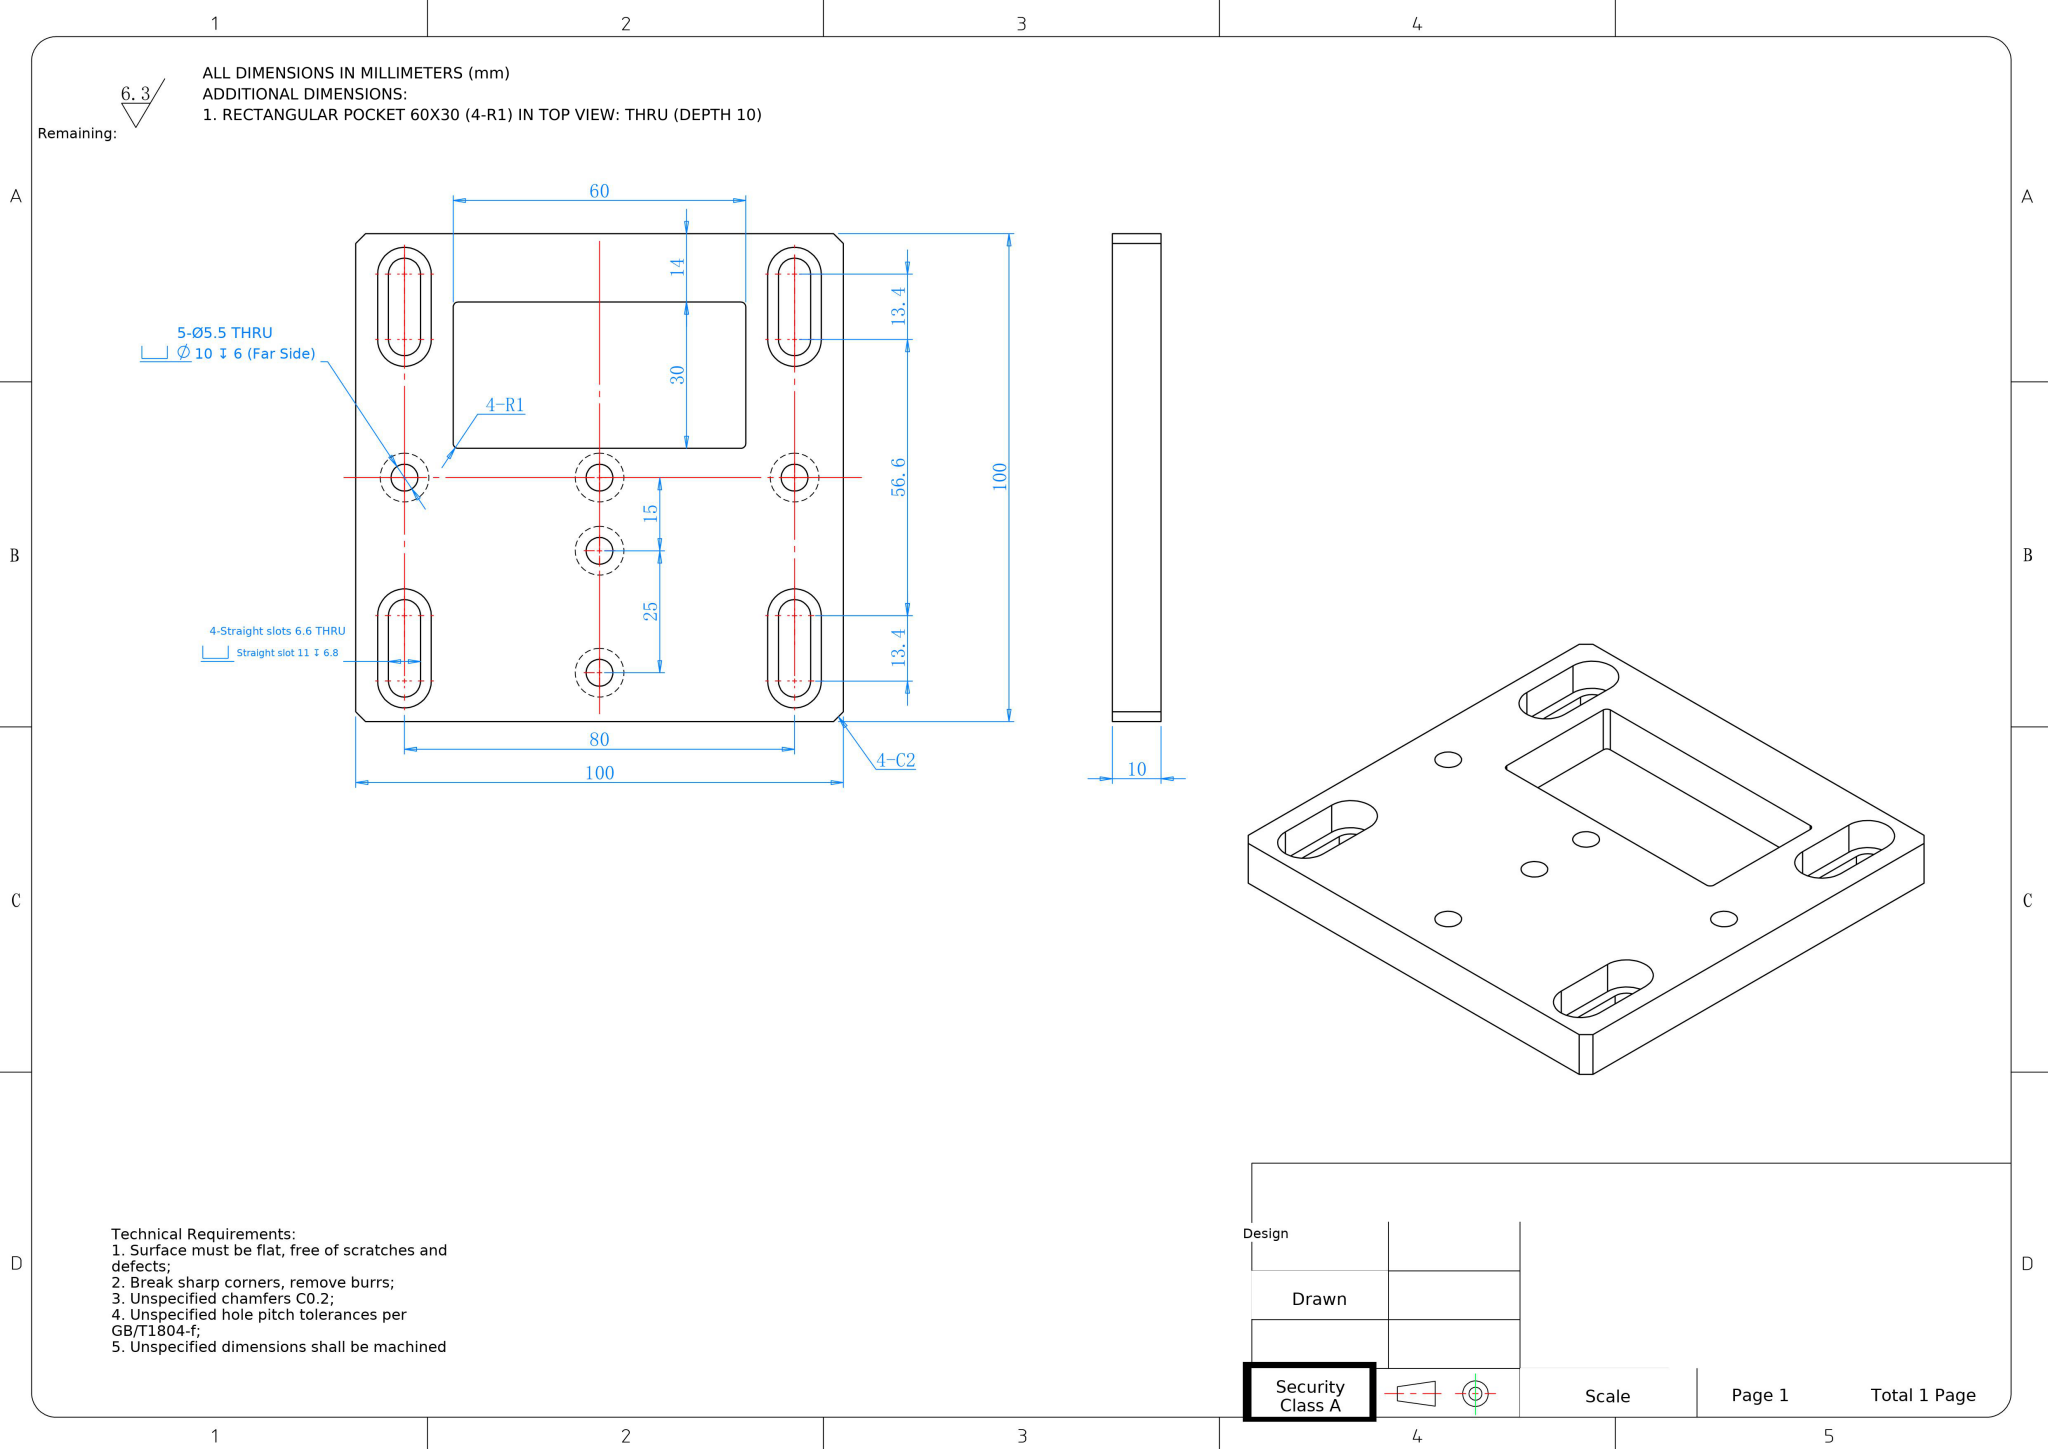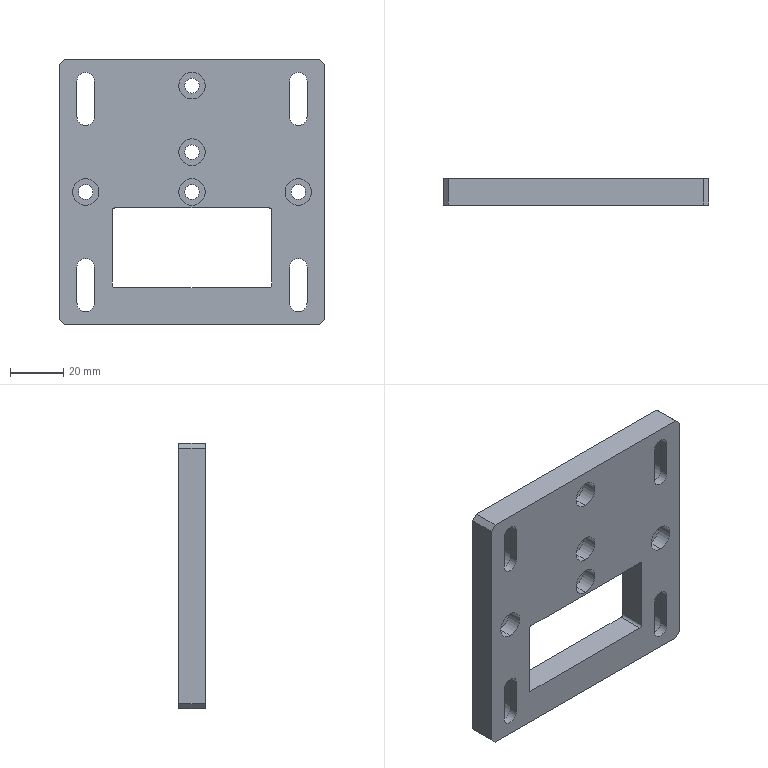Part | NX | mm | 1 solid | 87 faces | box 100 x 10 x 100 mm | volume 71015 mm3 | cylinder 48 | plane 39 | commonest cylinder face diameters 11 x12 6.6 x12 10 x10 5.5 x10 2 x4